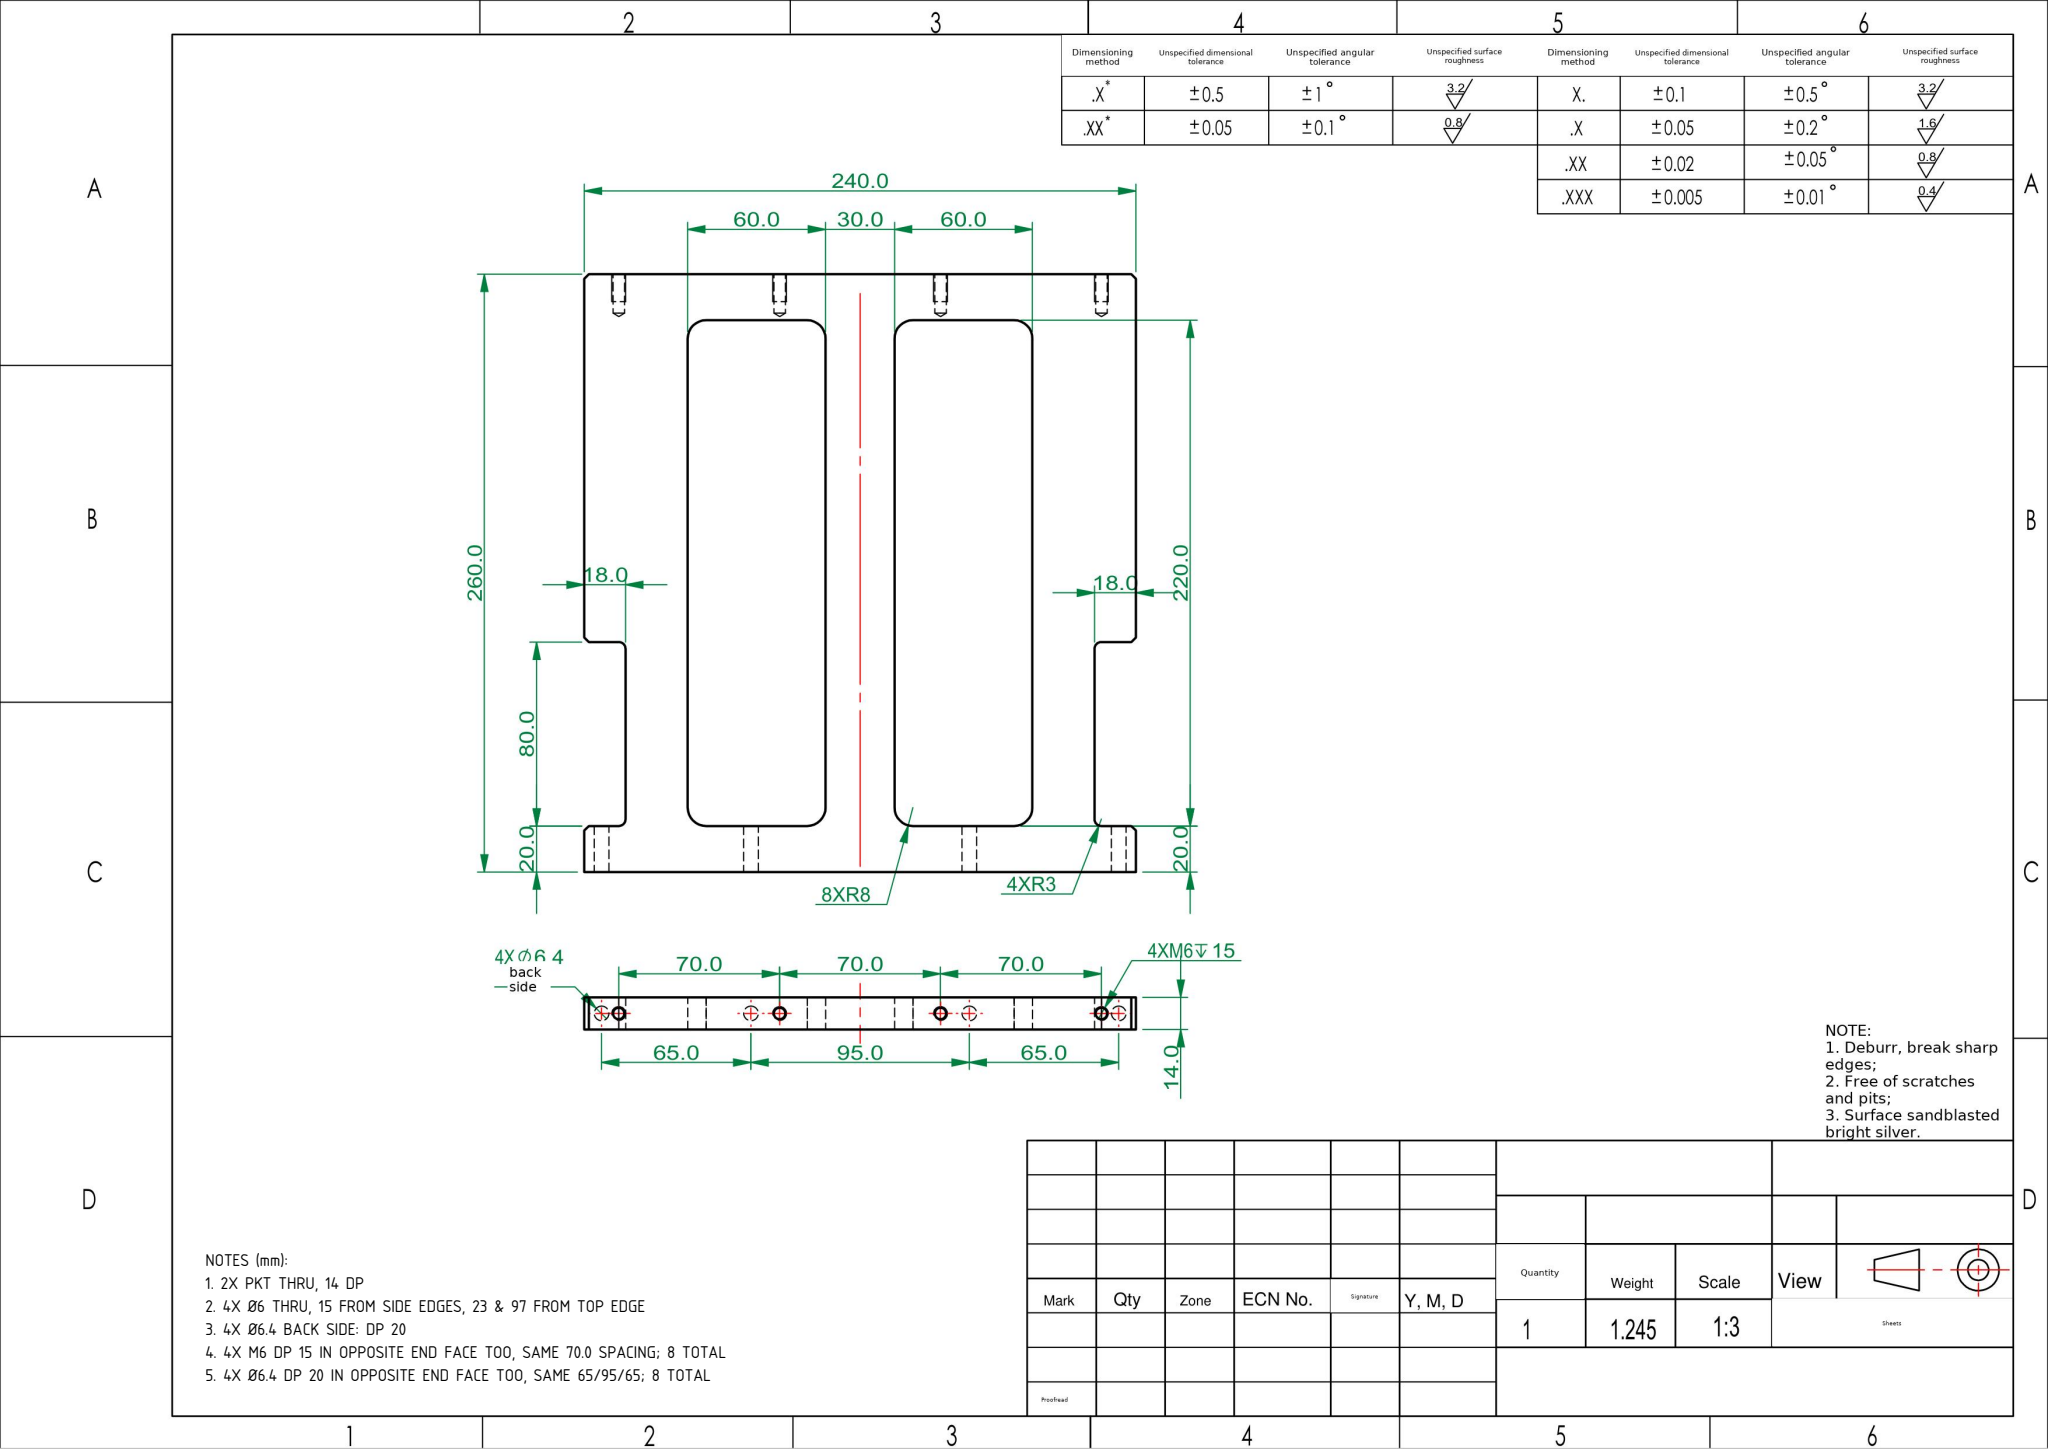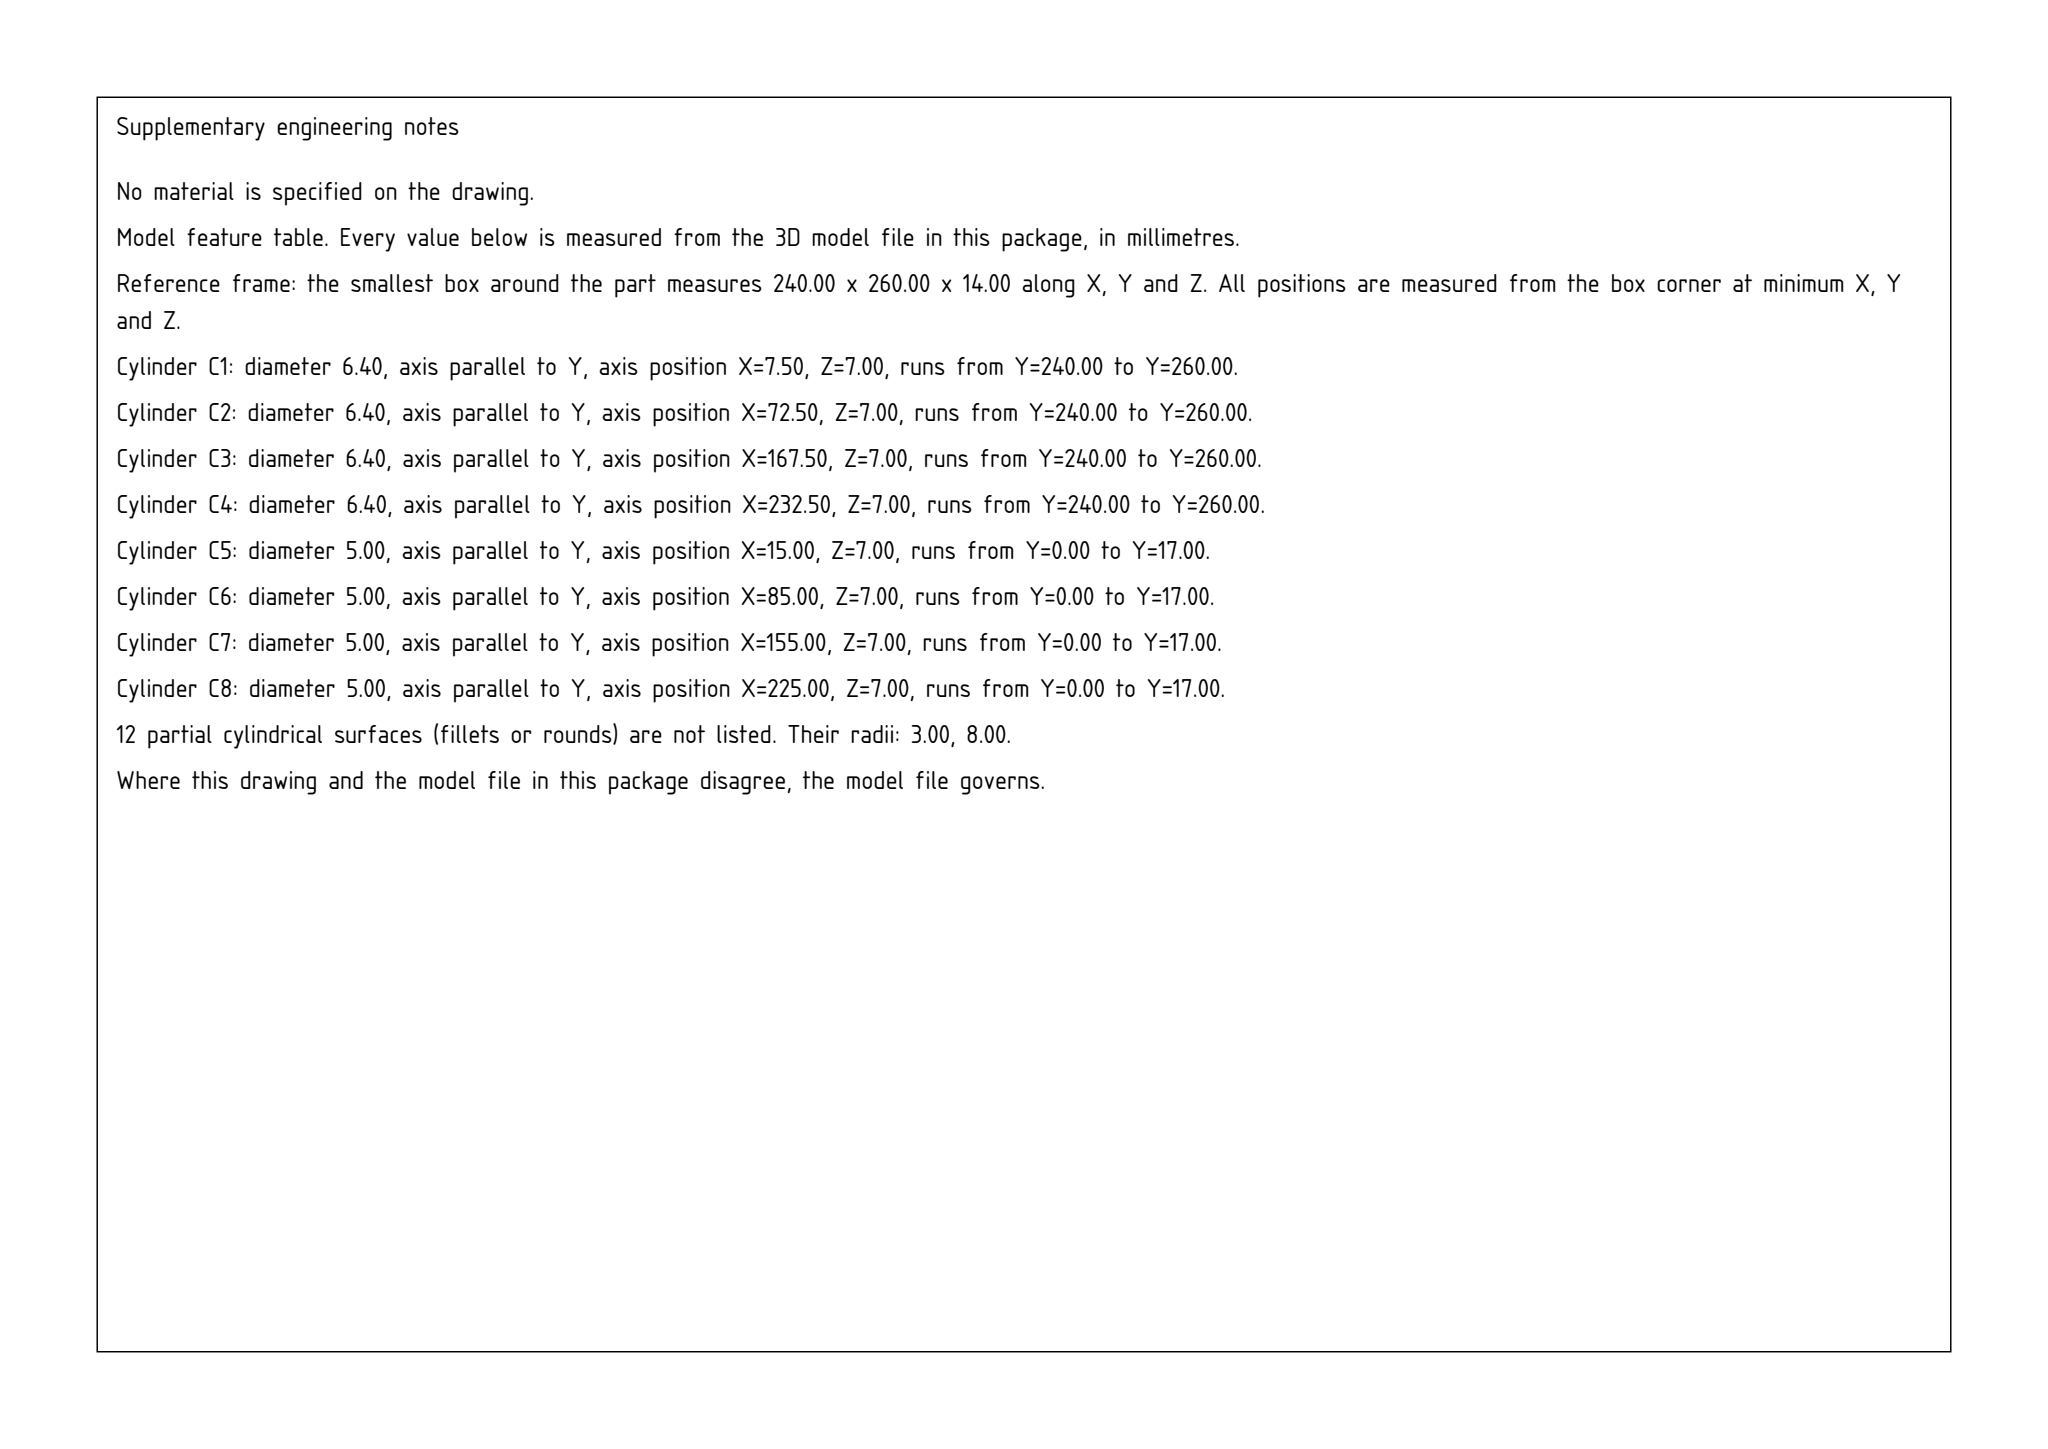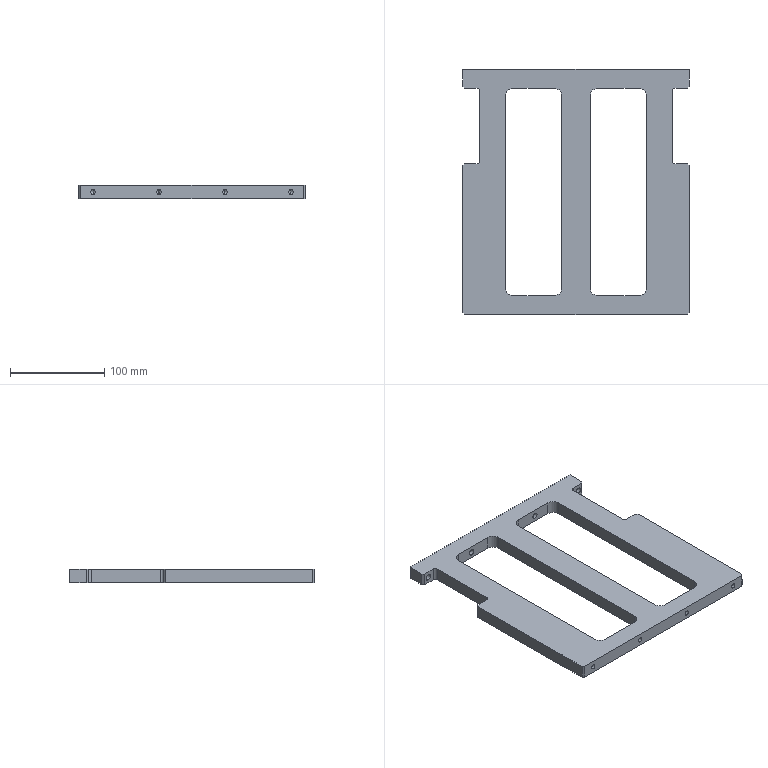Part | SolidWorks | mm | 1 solid | 64 faces | box 240 x 260 x 14 mm | volume 461210 mm3 | cylinder 28 | plane 28 | cone 8 | commonest cylinder face diameters 6.4 x8 5 x8 16 x8 6 x4
Drawing notes:
2X PKT THRU, 14 DP | from the solid: part z planes only 0 and 14; pocket corner cyls dia16 length 14 = full thickness
4X Ø6 THRU, 15 FROM SIDE EDGES, 23 & 97 FROM TOP EDGE | from the solid: dia6 z-axis cyls at (15,163)(15,237)(225,163)(225,237), length 14 thru; 260-237=23, 260-163=97
4X Ø6.4 BACK SIDE: DP 20 | from the solid: cyl dia 6.4, axis y, length 20.0 at z=7.0
4X M6 DP 15 IN OPPOSITE END FACE TOO, SAME 70.0 SPACING; 8 TOTAL | from the solid: dia 5.0 y-axis holes at x=15,85,155,225, z=7.0, count 2 each (both y faces)
4X Ø6.4 DP 20 IN OPPOSITE END FACE TOO, SAME 65/95/65; 8 TOTAL | from the solid: dia 6.4 y-axis holes at x=7.5,72.5,167.5,232.5, z=7.0, count 2 each (both y faces)
build123d program:
from build123d import *

# Parameters (mm, degrees)
SKETCH1_W                       = 240
SKETCH1_H                       = 260
BOSS_EXTRUDE1_DEPTH             = 14
M6_TAPPED_HOLE1_D               = 5
M6_TAPPED_HOLE1_DEPTH           = 17
M6_TAPPED_HOLE1_TIP             = 1.502
SKETCH4_W                       = 150
SKETCH4_H                       = 220
CUT_EXTRUDE1_DEPTH              = 135
SKETCH5_W                       = 30
SKETCH5_H                       = 220
BOSS_EXTRUDE2_DEPTH             = 14
SKETCH6_W                       = 18
SKETCH6_H                       = 80
CUT_EXTRUDE2_DEPTH              = 135
FILLET1_R                       = 8
F_6_4_6_4_DIAMETER_HOLE1_REACH  = 350.863
F_6_4_6_4_DIAMETER_HOLE1_BORE_R = 3.2
FILLET2_R                       = 3
CHAMFER1_SIZE                   = 2


with BuildPart() as part:
    # Sketch1 → Boss-Extrude1 (new body)
    with BuildSketch(Plane.XY):
        Rectangle(SKETCH1_W, SKETCH1_H)
    extrude(amount=BOSS_EXTRUDE1_DEPTH)

    # M6 Tapped Hole1
    with Locations(Plane(origin=(-105, -130, 7), x_dir=(0, 0, -1), z_dir=(0, -1, 0))):
        with Locations((0, 0), (0, 70), (0, 140), (0, 210)):
            Hole(M6_TAPPED_HOLE1_D / 2, depth=M6_TAPPED_HOLE1_DEPTH)
            with Locations((0, 0, -(M6_TAPPED_HOLE1_DEPTH + M6_TAPPED_HOLE1_TIP / 2))):  # 118° drill point
                Cone(0, M6_TAPPED_HOLE1_D / 2, M6_TAPPED_HOLE1_TIP, mode=Mode.SUBTRACT)

    # Sketch4 → Cut-Extrude1 (cut)
    with BuildSketch(Plane.XY.offset(14)):
        Rectangle(SKETCH4_W, SKETCH4_H)
    extrude(amount=-CUT_EXTRUDE1_DEPTH, mode=Mode.SUBTRACT)

    # Sketch5 → Boss-Extrude2 (add)
    with BuildSketch(Plane.XY.offset(14)):
        Rectangle(SKETCH5_W, SKETCH5_H)
    extrude(amount=-BOSS_EXTRUDE2_DEPTH)

    # Sketch6 → Cut-Extrude2 (cut)
    with BuildSketch(Plane(origin=(0, 0, 0), x_dir=(-1, 0, 0), z_dir=(0, 0, -1))):
        with Locations((-111, 70)):
            Rectangle(SKETCH6_W, SKETCH6_H)
        with Locations((111, 70)):
            Rectangle(SKETCH6_W, SKETCH6_H)
    extrude(amount=-CUT_EXTRUDE2_DEPTH, mode=Mode.SUBTRACT)

    # Fillet1
    fillet1_edges = [part.edges().sort_by_distance(p)[0] for p in [
        (75, 110, 7),
        (75, -110, 7),
        (-75, -110, 7),
        (-75, 110, 7),
        (15, 110, 7),
        (15, -110, 7),
        (-15, -110, 7),
        (-15, 110, 7),
    ]]
    fillet(fillet1_edges, radius=FILLET1_R)

    # 6.4 _6.4_ Diameter Hole1 bore (on position points) → 6.4 _6.4_ Diameter Hole1 (cut, up to next)
    with BuildSketch(Plane(origin=(-112.5, 130, 7), x_dir=(0, 0, 1), z_dir=(0, 1, 0)), mode=Mode.PRIVATE) as f_6_4_6_4_diameter_hole1_sk1:
        Circle(F_6_4_6_4_DIAMETER_HOLE1_BORE_R)
    f_6_4_6_4_diameter_hole1_tool1 = extrude(f_6_4_6_4_diameter_hole1_sk1.sketch, amount=-F_6_4_6_4_DIAMETER_HOLE1_REACH, mode=Mode.PRIVATE) & part.part
    # 6.4 _6.4_ Diameter Hole1 bore (on position points) → 6.4 _6.4_ Diameter Hole1 (cut, up to next)
    with BuildSketch(Plane(origin=(-112.5, 130, 7), x_dir=(0, 0, 1), z_dir=(0, 1, 0)), mode=Mode.PRIVATE) as f_6_4_6_4_diameter_hole1_sk2:
        with Locations((0, 65)):
            Circle(F_6_4_6_4_DIAMETER_HOLE1_BORE_R)
    f_6_4_6_4_diameter_hole1_tool2 = extrude(f_6_4_6_4_diameter_hole1_sk2.sketch, amount=-F_6_4_6_4_DIAMETER_HOLE1_REACH, mode=Mode.PRIVATE) & part.part
    # 6.4 _6.4_ Diameter Hole1 bore (on position points) → 6.4 _6.4_ Diameter Hole1 (cut, up to next)
    with BuildSketch(Plane(origin=(-112.5, 130, 7), x_dir=(0, 0, 1), z_dir=(0, 1, 0)), mode=Mode.PRIVATE) as f_6_4_6_4_diameter_hole1_sk3:
        with Locations((0, 160)):
            Circle(F_6_4_6_4_DIAMETER_HOLE1_BORE_R)
    f_6_4_6_4_diameter_hole1_tool3 = extrude(f_6_4_6_4_diameter_hole1_sk3.sketch, amount=-F_6_4_6_4_DIAMETER_HOLE1_REACH, mode=Mode.PRIVATE) & part.part
    # 6.4 _6.4_ Diameter Hole1 bore (on position points) → 6.4 _6.4_ Diameter Hole1 (cut, up to next)
    with BuildSketch(Plane(origin=(-112.5, 130, 7), x_dir=(0, 0, 1), z_dir=(0, 1, 0)), mode=Mode.PRIVATE) as f_6_4_6_4_diameter_hole1_sk4:
        with Locations((0, 225)):
            Circle(F_6_4_6_4_DIAMETER_HOLE1_BORE_R)
    f_6_4_6_4_diameter_hole1_tool4 = extrude(f_6_4_6_4_diameter_hole1_sk4.sketch, amount=-F_6_4_6_4_DIAMETER_HOLE1_REACH, mode=Mode.PRIVATE) & part.part
    add(f_6_4_6_4_diameter_hole1_tool1.solids().sort_by_distance((-112.5, 130, 7))[0], mode=Mode.SUBTRACT)
    add(f_6_4_6_4_diameter_hole1_tool2.solids().sort_by_distance((-47.5, 130, 7))[0], mode=Mode.SUBTRACT)
    add(f_6_4_6_4_diameter_hole1_tool3.solids().sort_by_distance((47.5, 130, 7))[0], mode=Mode.SUBTRACT)
    add(f_6_4_6_4_diameter_hole1_tool4.solids().sort_by_distance((112.5, 130, 7))[0], mode=Mode.SUBTRACT)

    # Fillet2
    fillet2_edges = [part.edges().sort_by_distance(p)[0] for p in [
        (102, 110, 7),
        (102, 30, 7),
        (-102, 30, 7),
        (-102, 110, 7),
    ]]
    fillet(fillet2_edges, radius=FILLET2_R)

    # Chamfer1
    chamfer1_edges = [part.edges().sort_by_distance(p)[0] for p in [
        (120, 30, 7),
        (120, 110, 7),
        (120, -130, 7),
        (-120, -130, 7),
        (-120, 110, 7),
        (-120, 30, 7),
    ]]
    chamfer(chamfer1_edges, length=CHAMFER1_SIZE)


solid = part.part